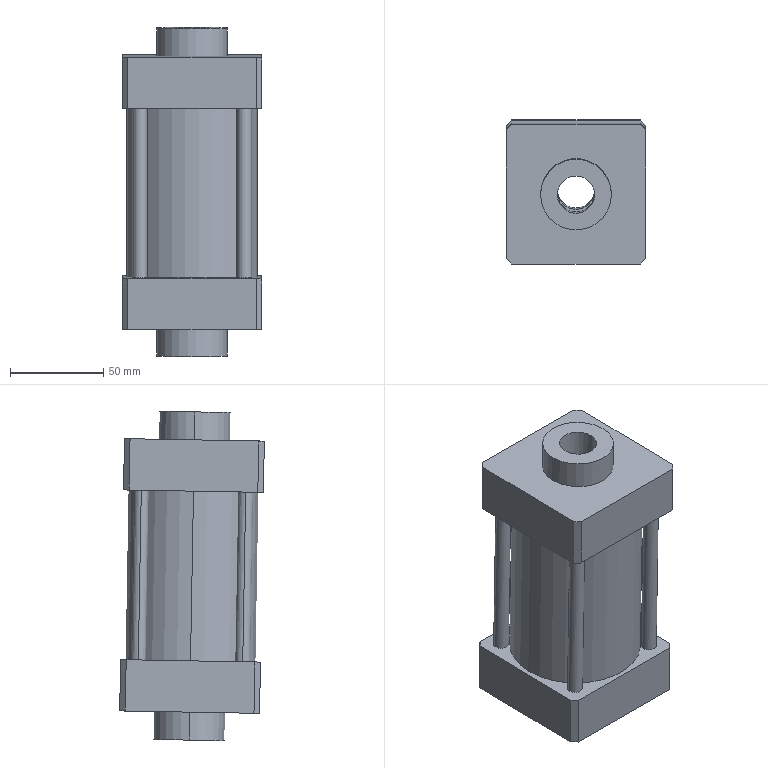Component | SolidWorks | SC63-50Cylinder-1 | 1 solid | 44 faces | volume 400541 mm3 | plane 24 | cylinder 20 | commonest cylinder face diameters 8 x8 38 x4 20 x4 63 x2 70 x2